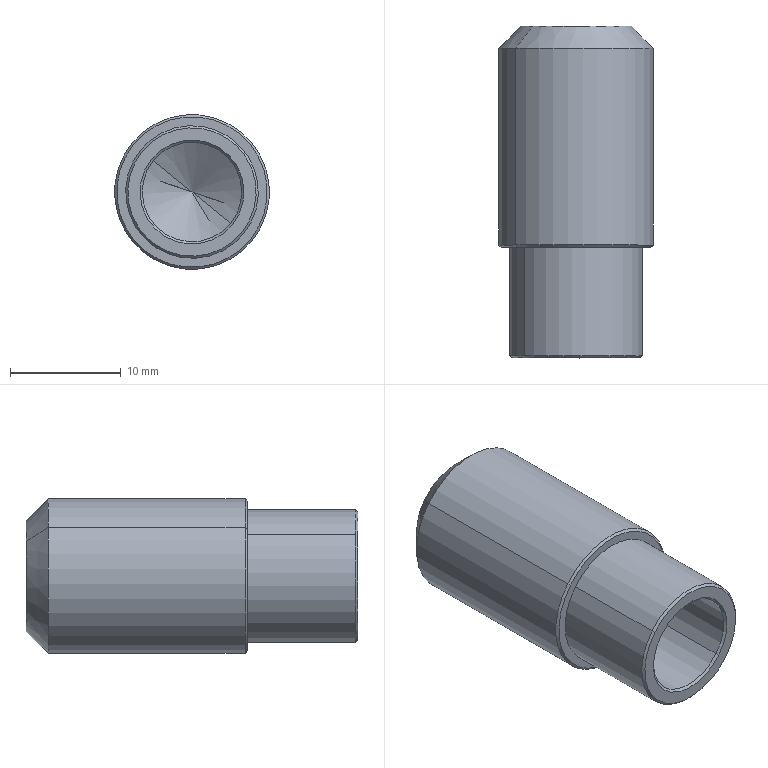Component | SolidWorks | GluePaperFeedingTensioningWheelAssembly-1_YX-04-114GluePaperFeedingTensioningWheelAdjustingPost-1 | 1 solid | 19 faces | box 14 x 30 x 14 mm | volume 2480 mm3 | cone 10 | cylinder 6 | plane 3 | commonest cylinder face diameters 12 x2 14 x2 9 x2 | material 45#Steel
build123d program:
from build123d import *


with BuildPart() as part:
    # Sketch1 → Revolve1 (revolve)
    with BuildSketch(Plane.XY, mode=Mode.PRIVATE) as revolve1_sk:
        Polygon((25, 4.5), (27.704, 0), (30, 0), (30, 5), (28, 7), (10.2, 7), (10, 6.8), (10, 6), (0.2, 6), (0, 5.8), (0, 4.7), (0.2, 4.5), align=None)
    revolve(revolve1_sk.sketch.rotate(Axis((0, 0, 0), (1, 0, 0)), 270), axis=Axis((0, 0, 0), (1, 0, 0)))


solid = part.part

# Placed as in the assembly
solid = solid.moved(Location((16.603, 31.262, 167), (0, 0, 90)))
STEP:
#1=CARTESIAN_POINT('',(0.7915,1.239,6.464));
#2=VERTEX_POINT('',#1);
#3=CARTESIAN_POINT('',(0.5158,1.239,6.686));
#4=VERTEX_POINT('',#3);
#5=CARTESIAN_POINT('',(0.6537,1.239,6.575));
#6=DIRECTION('',(-0.,1.,0.));
#7=DIRECTION('',(-0.778,0.,0.6282));
#8=AXIS2_PLACEMENT_3D('',#5,#6,#7);
#9=CIRCLE('',#8,0.1772);
#10=EDGE_CURVE('',#2,#4,#9,.T.);
#11=ORIENTED_EDGE('',*,*,#10,.T.);
#12=CARTESIAN_POINT('',(0.5097,1.231,6.691));
#13=VERTEX_POINT('',#12);
#14=CARTESIAN_POINT('',(0.5097,1.231,6.691));
#15=DIRECTION('',(-0.5501,-0.7071,0.4442));
#16=VECTOR('',#15,39.37);
#17=LINE('',#14,#16);
#18=EDGE_CURVE('',#4,#13,#17,.T.);
#19=ORIENTED_EDGE('',*,*,#18,.T.);
#20=CARTESIAN_POINT('',(0.7976,1.231,6.459));
#21=VERTEX_POINT('',#20);
#22=CARTESIAN_POINT('',(0.6537,1.231,6.575));
#23=DIRECTION('',(-0.,1.,0.));
#24=DIRECTION('',(-0.778,0.,0.6282));
#25=AXIS2_PLACEMENT_3D('',#22,#23,#24);
#26=CIRCLE('',#25,0.185);
#27=EDGE_CURVE('',#21,#13,#26,.T.);
#28=ORIENTED_EDGE('',*,*,#27,.F.);
#29=CARTESIAN_POINT('',(0.7976,1.231,6.459));
#30=DIRECTION('',(0.5501,-0.7071,-0.4442));
#31=VECTOR('',#30,39.37);
#32=LINE('',#29,#31);
#33=EDGE_CURVE('',#2,#21,#32,.T.);
#34=ORIENTED_EDGE('',*,*,#33,.F.);
#35=EDGE_LOOP('',(#11,#19,#28,#34));
#36=FACE_OUTER_BOUND('',#35,.T.);
#37=CARTESIAN_POINT('',(0.6537,1.231,6.575));
#38=DIRECTION('',(0.,-1.,-0.));
#39=DIRECTION('',(0.778,0.,-0.6282));
#40=AXIS2_PLACEMENT_3D('',#37,#38,#39);
#41=CONICAL_SURFACE('',#40,0.185,0.7854);
#42=ADVANCED_FACE('',(#36),#41,.F.);
#43=CARTESIAN_POINT('',(0.476,1.231,6.718));
#44=VERTEX_POINT('',#43);
#45=CARTESIAN_POINT('',(0.8313,1.231,6.431));
#46=VERTEX_POINT('',#45);
#47=CARTESIAN_POINT('',(0.6537,1.231,6.575));
#48=DIRECTION('',(-0.,1.,0.));
#49=DIRECTION('',(-0.778,0.,0.6282));
#50=AXIS2_PLACEMENT_3D('',#47,#48,#49);
#51=CIRCLE('',#50,0.2283);
#52=EDGE_CURVE('',#44,#46,#51,.T.);
#53=ORIENTED_EDGE('',*,*,#52,.T.);
#54=CARTESIAN_POINT('',(0.8374,1.239,6.426));
#55=VERTEX_POINT('',#54);
#56=CARTESIAN_POINT('',(0.8374,1.239,6.426));
#57=DIRECTION('',(0.5501,0.7071,-0.4442));
#58=VECTOR('',#57,39.37);
#59=LINE('',#56,#58);
#60=EDGE_CURVE('',#46,#55,#59,.T.);
#61=ORIENTED_EDGE('',*,*,#60,.T.);
#62=CARTESIAN_POINT('',(0.4699,1.239,6.723));
#63=VERTEX_POINT('',#62);
#64=CARTESIAN_POINT('',(0.6537,1.239,6.575));
#65=DIRECTION('',(-0.,1.,0.));
#66=DIRECTION('',(-0.778,0.,0.6282));
#67=AXIS2_PLACEMENT_3D('',#64,#65,#66);
#68=CIRCLE('',#67,0.2362);
#69=EDGE_CURVE('',#63,#55,#68,.T.);
#70=ORIENTED_EDGE('',*,*,#69,.F.);
#71=CARTESIAN_POINT('',(0.4699,1.239,6.723));
#72=DIRECTION('',(-0.5501,0.7071,0.4442));
#73=VECTOR('',#72,39.37);
#74=LINE('',#71,#73);
#75=EDGE_CURVE('',#44,#63,#74,.T.);
#76=ORIENTED_EDGE('',*,*,#75,.F.);
#77=EDGE_LOOP('',(#53,#61,#70,#76));
#78=FACE_OUTER_BOUND('',#77,.T.);
#79=CARTESIAN_POINT('',(0.6537,1.239,6.575));
#80=DIRECTION('',(-0.,1.,0.));
#81=DIRECTION('',(-0.778,0.,0.6282));
#82=AXIS2_PLACEMENT_3D('',#79,#80,#81);
#83=CONICAL_SURFACE('',#82,0.2362,0.7854);
#84=ADVANCED_FACE('',(#78),#83,.T.);
#85=ORIENTED_EDGE('',*,*,#69,.T.);
#86=CARTESIAN_POINT('',(0.8374,1.624,6.426));
#87=VERTEX_POINT('',#86);
#88=CARTESIAN_POINT('',(0.8374,1.231,6.426));
#89=DIRECTION('',(-0.,1.,0.));
#90=VECTOR('',#89,39.37);
#91=LINE('',#88,#90);
#92=EDGE_CURVE('',#55,#87,#91,.T.);
#93=ORIENTED_EDGE('',*,*,#92,.T.);
#94=CARTESIAN_POINT('',(0.4699,1.624,6.723));
#95=VERTEX_POINT('',#94);
#96=CARTESIAN_POINT('',(0.6537,1.624,6.575));
#97=DIRECTION('',(-0.,1.,0.));
#98=DIRECTION('',(-0.778,0.,0.6282));
#99=AXIS2_PLACEMENT_3D('',#96,#97,#98);
#100=CIRCLE('',#99,0.2362);
#101=EDGE_CURVE('',#95,#87,#100,.T.);
#102=ORIENTED_EDGE('',*,*,#101,.F.);
#103=CARTESIAN_POINT('',(0.4699,1.231,6.723));
#104=DIRECTION('',(-0.,1.,0.));
#105=VECTOR('',#104,39.37);
#106=LINE('',#103,#105);
#107=EDGE_CURVE('',#63,#95,#106,.T.);
#108=ORIENTED_EDGE('',*,*,#107,.F.);
#109=EDGE_LOOP('',(#85,#93,#102,#108));
#110=FACE_OUTER_BOUND('',#109,.T.);
#111=CARTESIAN_POINT('',(0.6537,1.231,6.575));
#112=DIRECTION('',(-0.,1.,0.));
#113=DIRECTION('',(-0.778,0.,0.6282));
#114=AXIS2_PLACEMENT_3D('',#111,#112,#113);
#115=CYLINDRICAL_SURFACE('',#114,0.2362);
#116=ADVANCED_FACE('',(#110),#115,.T.);
#117=CARTESIAN_POINT('',(0.4454,1.624,6.743));
#118=VERTEX_POINT('',#117);
#119=CARTESIAN_POINT('',(0.8619,1.624,6.407));
#120=VERTEX_POINT('',#119);
#121=CARTESIAN_POINT('',(0.6537,1.624,6.575));
#122=DIRECTION('',(-0.,1.,0.));
#123=DIRECTION('',(-0.778,0.,0.6282));
#124=AXIS2_PLACEMENT_3D('',#121,#122,#123);
#125=CIRCLE('',#124,0.2677);
#126=EDGE_CURVE('',#118,#120,#125,.T.);
#127=ORIENTED_EDGE('',*,*,#126,.T.);
#128=CARTESIAN_POINT('',(0.8681,1.632,6.402));
#129=VERTEX_POINT('',#128);
#130=CARTESIAN_POINT('',(0.8681,1.632,6.402));
#131=DIRECTION('',(0.5501,0.7071,-0.4442));
#132=VECTOR('',#131,39.37);
#133=LINE('',#130,#132);
#134=EDGE_CURVE('',#120,#129,#133,.T.);
#135=ORIENTED_EDGE('',*,*,#134,.T.);
#136=CARTESIAN_POINT('',(0.4392,1.632,6.748));
#137=VERTEX_POINT('',#136);
#138=CARTESIAN_POINT('',(0.6537,1.632,6.575));
#139=DIRECTION('',(-0.,1.,0.));
#140=DIRECTION('',(-0.778,0.,0.6282));
#141=AXIS2_PLACEMENT_3D('',#138,#139,#140);
#142=CIRCLE('',#141,0.2756);
#143=EDGE_CURVE('',#137,#129,#142,.T.);
#144=ORIENTED_EDGE('',*,*,#143,.F.);
#145=CARTESIAN_POINT('',(0.4392,1.632,6.748));
#146=DIRECTION('',(-0.5501,0.7071,0.4442));
#147=VECTOR('',#146,39.37);
#148=LINE('',#145,#147);
#149=EDGE_CURVE('',#118,#137,#148,.T.);
#150=ORIENTED_EDGE('',*,*,#149,.F.);
#151=EDGE_LOOP('',(#127,#135,#144,#150));
#152=FACE_OUTER_BOUND('',#151,.T.);
#153=CARTESIAN_POINT('',(0.6537,1.632,6.575));
#154=DIRECTION('',(-0.,1.,0.));
#155=DIRECTION('',(-0.778,0.,0.6282));
#156=AXIS2_PLACEMENT_3D('',#153,#154,#155);
#157=CONICAL_SURFACE('',#156,0.2756,0.7854);
#158=ADVANCED_FACE('',(#152),#157,.T.);
#159=ORIENTED_EDGE('',*,*,#143,.T.);
#160=CARTESIAN_POINT('',(0.8681,2.333,6.402));
#161=VERTEX_POINT('',#160);
#162=CARTESIAN_POINT('',(0.8681,1.231,6.402));
#163=DIRECTION('',(-0.,1.,0.));
#164=VECTOR('',#163,39.37);
#165=LINE('',#162,#164);
#166=EDGE_CURVE('',#129,#161,#165,.T.);
#167=ORIENTED_EDGE('',*,*,#166,.T.);
#168=CARTESIAN_POINT('',(0.4392,2.333,6.748));
#169=VERTEX_POINT('',#168);
#170=CARTESIAN_POINT('',(0.6537,2.333,6.575));
#171=DIRECTION('',(-0.,1.,0.));
#172=DIRECTION('',(-0.778,0.,0.6282));
#173=AXIS2_PLACEMENT_3D('',#170,#171,#172);
#174=CIRCLE('',#173,0.2756);
#175=EDGE_CURVE('',#169,#161,#174,.T.);
#176=ORIENTED_EDGE('',*,*,#175,.F.);
#177=CARTESIAN_POINT('',(0.4392,1.231,6.748));
#178=DIRECTION('',(-0.,1.,0.));
#179=VECTOR('',#178,39.37);
#180=LINE('',#177,#179);
#181=EDGE_CURVE('',#137,#169,#180,.T.);
#182=ORIENTED_EDGE('',*,*,#181,.F.);
#183=EDGE_LOOP('',(#159,#167,#176,#182));
#184=FACE_OUTER_BOUND('',#183,.T.);
#185=CARTESIAN_POINT('',(0.6537,1.231,6.575));
#186=DIRECTION('',(-0.,1.,0.));
#187=DIRECTION('',(-0.778,0.,0.6282));
#188=AXIS2_PLACEMENT_3D('',#185,#186,#187);
#189=CYLINDRICAL_SURFACE('',#188,0.2756);
#190=ADVANCED_FACE('',(#184),#189,.T.);
#191=CARTESIAN_POINT('',(0.5005,2.412,6.698));
#192=VERTEX_POINT('',#191);
#193=CARTESIAN_POINT('',(0.8068,2.412,6.451));
#194=VERTEX_POINT('',#193);
#195=CARTESIAN_POINT('',(0.6537,2.412,6.575));
#196=DIRECTION('',(-0.,1.,0.));
#197=DIRECTION('',(-0.778,0.,0.6282));
#198=AXIS2_PLACEMENT_3D('',#195,#196,#197);
#199=CIRCLE('',#198,0.1969);
#200=EDGE_CURVE('',#192,#194,#199,.T.);
#201=ORIENTED_EDGE('',*,*,#200,.F.);
#202=CARTESIAN_POINT('',(0.5005,2.412,6.698));
#203=DIRECTION('',(-0.5501,-0.7071,0.4442));
#204=VECTOR('',#203,39.37);
#205=LINE('',#202,#204);
#206=EDGE_CURVE('',#192,#169,#205,.T.);
#207=ORIENTED_EDGE('',*,*,#206,.T.);
#208=ORIENTED_EDGE('',*,*,#175,.T.);
#209=CARTESIAN_POINT('',(0.8068,2.412,6.451));
#210=DIRECTION('',(0.5501,-0.7071,-0.4442));
#211=VECTOR('',#210,39.37);
#212=LINE('',#209,#211);
#213=EDGE_CURVE('',#194,#161,#212,.T.);
#214=ORIENTED_EDGE('',*,*,#213,.F.);
#215=EDGE_LOOP('',(#201,#207,#208,#214));
#216=FACE_OUTER_BOUND('',#215,.T.);
#217=CARTESIAN_POINT('',(0.6537,2.412,6.575));
#218=DIRECTION('',(0.,-1.,-0.));
#219=DIRECTION('',(0.778,0.,-0.6282));
#220=AXIS2_PLACEMENT_3D('',#217,#218,#219);
#221=CONICAL_SURFACE('',#220,0.1969,0.7854);
#222=ADVANCED_FACE('',(#216),#221,.T.);
#223=CARTESIAN_POINT('',(0.6537,2.321,6.575));
#224=VERTEX_POINT('',#223);
#225=CARTESIAN_POINT('',(0.7915,2.215,6.464));
#226=VERTEX_POINT('',#225);
#227=CARTESIAN_POINT('',(0.7915,2.215,6.464));
#228=DIRECTION('',(0.6669,-0.515,-0.5385));
#229=VECTOR('',#228,39.37);
#230=LINE('',#227,#229);
#231=EDGE_CURVE('',#224,#226,#230,.T.);
#232=ORIENTED_EDGE('',*,*,#231,.F.);
#233=CARTESIAN_POINT('',(0.5158,2.215,6.686));
#234=VERTEX_POINT('',#233);
#235=CARTESIAN_POINT('',(0.5158,2.215,6.686));
#236=DIRECTION('',(-0.6669,-0.515,0.5385));
#237=VECTOR('',#236,39.37);
#238=LINE('',#235,#237);
#239=EDGE_CURVE('',#224,#234,#238,.T.);
#240=ORIENTED_EDGE('',*,*,#239,.T.);
#241=CARTESIAN_POINT('',(0.6537,2.215,6.575));
#242=DIRECTION('',(-0.,1.,0.));
#243=DIRECTION('',(-0.778,0.,0.6282));
#244=AXIS2_PLACEMENT_3D('',#241,#242,#243);
#245=CIRCLE('',#244,0.1772);
#246=EDGE_CURVE('',#226,#234,#245,.T.);
#247=ORIENTED_EDGE('',*,*,#246,.F.);
#248=EDGE_LOOP('',(#232,#240,#247));
#249=FACE_OUTER_BOUND('',#248,.T.);
#250=CARTESIAN_POINT('',(0.6537,2.215,6.575));
#251=DIRECTION('',(0.,-1.,-0.));
#252=DIRECTION('',(0.778,0.,-0.6282));
#253=AXIS2_PLACEMENT_3D('',#250,#251,#252);
#254=CONICAL_SURFACE('',#253,0.1772,1.03);
#255=ADVANCED_FACE('',(#249),#254,.F.);
#256=ORIENTED_EDGE('',*,*,#10,.F.);
#257=CARTESIAN_POINT('',(0.7915,1.231,6.464));
#258=DIRECTION('',(-0.,1.,0.));
#259=VECTOR('',#258,39.37);
#260=LINE('',#257,#259);
#261=EDGE_CURVE('',#2,#226,#260,.T.);
#262=ORIENTED_EDGE('',*,*,#261,.T.);
#263=ORIENTED_EDGE('',*,*,#246,.T.);
#264=CARTESIAN_POINT('',(0.5158,1.231,6.686));
#265=DIRECTION('',(-0.,1.,0.));
#266=VECTOR('',#265,39.37);
#267=LINE('',#264,#266);
#268=EDGE_CURVE('',#4,#234,#267,.T.);
#269=ORIENTED_EDGE('',*,*,#268,.F.);
#270=EDGE_LOOP('',(#256,#262,#263,#269));
#271=FACE_OUTER_BOUND('',#270,.T.);
#272=CARTESIAN_POINT('',(0.6537,1.231,6.575));
#273=DIRECTION('',(-0.,1.,0.));
#274=DIRECTION('',(-0.778,0.,0.6282));
#275=AXIS2_PLACEMENT_3D('',#272,#273,#274);
#276=CYLINDRICAL_SURFACE('',#275,0.1772);
#277=ADVANCED_FACE('',(#271),#276,.F.);
#278=ORIENTED_EDGE('',*,*,#261,.F.);
#279=CARTESIAN_POINT('',(0.6537,1.239,6.575));
#280=DIRECTION('',(-0.,1.,0.));
#281=DIRECTION('',(-0.778,0.,0.6282));
#282=AXIS2_PLACEMENT_3D('',#279,#280,#281);
#283=CIRCLE('',#282,0.1772);
#284=EDGE_CURVE('',#4,#2,#283,.T.);
#285=ORIENTED_EDGE('',*,*,#284,.F.);
#286=ORIENTED_EDGE('',*,*,#268,.T.);
#287=CARTESIAN_POINT('',(0.6537,2.215,6.575));
#288=DIRECTION('',(-0.,1.,0.));
#289=DIRECTION('',(-0.778,0.,0.6282));
#290=AXIS2_PLACEMENT_3D('',#287,#288,#289);
#291=CIRCLE('',#290,0.1772);
#292=EDGE_CURVE('',#234,#226,#291,.T.);
#293=ORIENTED_EDGE('',*,*,#292,.T.);
#294=EDGE_LOOP('',(#278,#285,#286,#293));
#295=FACE_OUTER_BOUND('',#294,.T.);
#296=CARTESIAN_POINT('',(0.6537,1.231,6.575));
#297=DIRECTION('',(-0.,1.,0.));
#298=DIRECTION('',(-0.778,0.,0.6282));
#299=AXIS2_PLACEMENT_3D('',#296,#297,#298);
#300=CYLINDRICAL_SURFACE('',#299,0.1772);
#301=ADVANCED_FACE('',(#295),#300,.F.);
#302=ORIENTED_EDGE('',*,*,#239,.F.);
#303=ORIENTED_EDGE('',*,*,#231,.T.);
#304=ORIENTED_EDGE('',*,*,#292,.F.);
#305=EDGE_LOOP('',(#302,#303,#304));
#306=FACE_OUTER_BOUND('',#305,.T.);
#307=CARTESIAN_POINT('',(0.6537,2.215,6.575));
#308=DIRECTION('',(0.,-1.,-0.));
#309=DIRECTION('',(0.778,0.,-0.6282));
#310=AXIS2_PLACEMENT_3D('',#307,#308,#309);
#311=CONICAL_SURFACE('',#310,0.1772,1.03);
#312=ADVANCED_FACE('',(#306),#311,.F.);
#313=CARTESIAN_POINT('',(0.6537,2.412,6.575));
#314=DIRECTION('',(-0.,1.,0.));
#315=DIRECTION('',(-0.778,0.,0.6282));
#316=AXIS2_PLACEMENT_3D('',#313,#314,#315);
#317=CIRCLE('',#316,0.1969);
#318=EDGE_CURVE('',#194,#192,#317,.T.);
#319=ORIENTED_EDGE('',*,*,#318,.T.);
#320=ORIENTED_EDGE('',*,*,#200,.T.);
#321=EDGE_LOOP('',(#319,#320));
#322=FACE_OUTER_BOUND('',#321,.T.);
#323=CARTESIAN_POINT('',(0.6537,2.412,6.575));
#324=DIRECTION('',(-0.,1.,0.));
#325=DIRECTION('',(-0.778,-0.,0.6282));
#326=AXIS2_PLACEMENT_3D('',#323,#324,#325);
#327=PLANE('',#326);
#328=ADVANCED_FACE('',(#322),#327,.T.);
#329=ORIENTED_EDGE('',*,*,#206,.F.);
#330=ORIENTED_EDGE('',*,*,#318,.F.);
#331=ORIENTED_EDGE('',*,*,#213,.T.);
#332=CARTESIAN_POINT('',(0.6537,2.333,6.575));
#333=DIRECTION('',(-0.,1.,0.));
#334=DIRECTION('',(-0.778,0.,0.6282));
#335=AXIS2_PLACEMENT_3D('',#332,#333,#334);
#336=CIRCLE('',#335,0.2756);
#337=EDGE_CURVE('',#161,#169,#336,.T.);
#338=ORIENTED_EDGE('',*,*,#337,.T.);
#339=EDGE_LOOP('',(#329,#330,#331,#338));
#340=FACE_OUTER_BOUND('',#339,.T.);
#341=CARTESIAN_POINT('',(0.6537,2.412,6.575));
#342=DIRECTION('',(0.,-1.,-0.));
#343=DIRECTION('',(0.778,0.,-0.6282));
#344=AXIS2_PLACEMENT_3D('',#341,#342,#343);
#345=CONICAL_SURFACE('',#344,0.1969,0.7854);
#346=ADVANCED_FACE('',(#340),#345,.T.);
#347=ORIENTED_EDGE('',*,*,#166,.F.);
#348=CARTESIAN_POINT('',(0.6537,1.632,6.575));
#349=DIRECTION('',(-0.,1.,0.));
#350=DIRECTION('',(-0.778,0.,0.6282));
#351=AXIS2_PLACEMENT_3D('',#348,#349,#350);
#352=CIRCLE('',#351,0.2756);
#353=EDGE_CURVE('',#129,#137,#352,.T.);
#354=ORIENTED_EDGE('',*,*,#353,.T.);
#355=ORIENTED_EDGE('',*,*,#181,.T.);
#356=ORIENTED_EDGE('',*,*,#337,.F.);
#357=EDGE_LOOP('',(#347,#354,#355,#356));
#358=FACE_OUTER_BOUND('',#357,.T.);
#359=CARTESIAN_POINT('',(0.6537,1.231,6.575));
#360=DIRECTION('',(-0.,1.,0.));
#361=DIRECTION('',(-0.778,0.,0.6282));
#362=AXIS2_PLACEMENT_3D('',#359,#360,#361);
#363=CYLINDRICAL_SURFACE('',#362,0.2756);
#364=ADVANCED_FACE('',(#358),#363,.T.);
#365=ORIENTED_EDGE('',*,*,#134,.F.);
#366=CARTESIAN_POINT('',(0.6537,1.624,6.575));
#367=DIRECTION('',(-0.,1.,0.));
#368=DIRECTION('',(-0.778,0.,0.6282));
#369=AXIS2_PLACEMENT_3D('',#366,#367,#368);
#370=CIRCLE('',#369,0.2677);
#371=EDGE_CURVE('',#120,#118,#370,.T.);
#372=ORIENTED_EDGE('',*,*,#371,.T.);
#373=ORIENTED_EDGE('',*,*,#149,.T.);
#374=ORIENTED_EDGE('',*,*,#353,.F.);
#375=EDGE_LOOP('',(#365,#372,#373,#374));
#376=FACE_OUTER_BOUND('',#375,.T.);
#377=CARTESIAN_POINT('',(0.6537,1.632,6.575));
#378=DIRECTION('',(-0.,1.,0.));
#379=DIRECTION('',(-0.778,0.,0.6282));
#380=AXIS2_PLACEMENT_3D('',#377,#378,#379);
#381=CONICAL_SURFACE('',#380,0.2756,0.7854);
#382=ADVANCED_FACE('',(#376),#381,.T.);
#383=ORIENTED_EDGE('',*,*,#101,.T.);
#384=CARTESIAN_POINT('',(0.6537,1.624,6.575));
#385=DIRECTION('',(-0.,1.,0.));
#386=DIRECTION('',(-0.778,0.,0.6282));
#387=AXIS2_PLACEMENT_3D('',#384,#385,#386);
#388=CIRCLE('',#387,0.2362);
#389=EDGE_CURVE('',#87,#95,#388,.T.);
#390=ORIENTED_EDGE('',*,*,#389,.T.);
#391=EDGE_LOOP('',(#383,#390));
#392=FACE_BOUND('',#391,.T.);
#393=ORIENTED_EDGE('',*,*,#126,.F.);
#394=ORIENTED_EDGE('',*,*,#371,.F.);
#395=EDGE_LOOP('',(#393,#394));
#396=FACE_OUTER_BOUND('',#395,.T.);
#397=CARTESIAN_POINT('',(0.8218,1.624,6.783));
#398=DIRECTION('',(0.,-1.,-0.));
#399=DIRECTION('',(0.778,0.,-0.6282));
#400=AXIS2_PLACEMENT_3D('',#397,#398,#399);
#401=PLANE('',#400);
#402=ADVANCED_FACE('',(#392,#396),#401,.T.);
#403=ORIENTED_EDGE('',*,*,#92,.F.);
#404=CARTESIAN_POINT('',(0.6537,1.239,6.575));
#405=DIRECTION('',(-0.,1.,0.));
#406=DIRECTION('',(-0.778,0.,0.6282));
#407=AXIS2_PLACEMENT_3D('',#404,#405,#406);
#408=CIRCLE('',#407,0.2362);
#409=EDGE_CURVE('',#55,#63,#408,.T.);
#410=ORIENTED_EDGE('',*,*,#409,.T.);
#411=ORIENTED_EDGE('',*,*,#107,.T.);
#412=ORIENTED_EDGE('',*,*,#389,.F.);
#413=EDGE_LOOP('',(#403,#410,#411,#412));
#414=FACE_OUTER_BOUND('',#413,.T.);
#415=CARTESIAN_POINT('',(0.6537,1.231,6.575));
#416=DIRECTION('',(-0.,1.,0.));
#417=DIRECTION('',(-0.778,0.,0.6282));
#418=AXIS2_PLACEMENT_3D('',#415,#416,#417);
#419=CYLINDRICAL_SURFACE('',#418,0.2362);
#420=ADVANCED_FACE('',(#414),#419,.T.);
#421=ORIENTED_EDGE('',*,*,#60,.F.);
#422=CARTESIAN_POINT('',(0.6537,1.231,6.575));
#423=DIRECTION('',(-0.,1.,0.));
#424=DIRECTION('',(-0.778,0.,0.6282));
#425=AXIS2_PLACEMENT_3D('',#422,#423,#424);
#426=CIRCLE('',#425,0.2283);
#427=EDGE_CURVE('',#46,#44,#426,.T.);
#428=ORIENTED_EDGE('',*,*,#427,.T.);
#429=ORIENTED_EDGE('',*,*,#75,.T.);
#430=ORIENTED_EDGE('',*,*,#409,.F.);
#431=EDGE_LOOP('',(#421,#428,#429,#430));
#432=FACE_OUTER_BOUND('',#431,.T.);
#433=CARTESIAN_POINT('',(0.6537,1.239,6.575));
#434=DIRECTION('',(-0.,1.,0.));
#435=DIRECTION('',(-0.778,0.,0.6282));
#436=AXIS2_PLACEMENT_3D('',#433,#434,#435);
#437=CONICAL_SURFACE('',#436,0.2362,0.7854);
#438=ADVANCED_FACE('',(#432),#437,.T.);
#439=ORIENTED_EDGE('',*,*,#27,.T.);
#440=CARTESIAN_POINT('',(0.6537,1.231,6.575));
#441=DIRECTION('',(-0.,1.,0.));
#442=DIRECTION('',(-0.778,0.,0.6282));
#443=AXIS2_PLACEMENT_3D('',#440,#441,#442);
#444=CIRCLE('',#443,0.185);
#445=EDGE_CURVE('',#13,#21,#444,.T.);
#446=ORIENTED_EDGE('',*,*,#445,.T.);
#447=EDGE_LOOP('',(#439,#446));
#448=FACE_BOUND('',#447,.T.);
#449=ORIENTED_EDGE('',*,*,#52,.F.);
#450=ORIENTED_EDGE('',*,*,#427,.F.);
#451=EDGE_LOOP('',(#449,#450));
#452=FACE_OUTER_BOUND('',#451,.T.);
#453=CARTESIAN_POINT('',(0.7971,1.231,6.752));
#454=DIRECTION('',(0.,-1.,-0.));
#455=DIRECTION('',(0.778,0.,-0.6282));
#456=AXIS2_PLACEMENT_3D('',#453,#454,#455);
#457=PLANE('',#456);
#458=ADVANCED_FACE('',(#448,#452),#457,.T.);
#459=ORIENTED_EDGE('',*,*,#18,.F.);
#460=ORIENTED_EDGE('',*,*,#284,.T.);
#461=ORIENTED_EDGE('',*,*,#33,.T.);
#462=ORIENTED_EDGE('',*,*,#445,.F.);
#463=EDGE_LOOP('',(#459,#460,#461,#462));
#464=FACE_OUTER_BOUND('',#463,.T.);
#465=CARTESIAN_POINT('',(0.6537,1.231,6.575));
#466=DIRECTION('',(0.,-1.,-0.));
#467=DIRECTION('',(0.778,0.,-0.6282));
#468=AXIS2_PLACEMENT_3D('',#465,#466,#467);
#469=CONICAL_SURFACE('',#468,0.185,0.7854);
#470=ADVANCED_FACE('',(#464),#469,.F.);
#471=CLOSED_SHELL('',(#42,#84,#116,#158,#190,#222,#255,#277,#301,#312,#328,#346,#364,#382,#402,#420,#438,#458,#470));
#472=MANIFOLD_SOLID_BREP('',#471);
#473=CARTESIAN_POINT('',(0.,0.,0.));
#474=DIRECTION('',(0.,0.,1.));
#475=DIRECTION('',(1.,0.,0.));
#476=AXIS2_PLACEMENT_3D('',#473,#474,#475);
#477=(LENGTH_UNIT()NAMED_UNIT(*)SI_UNIT($,.METRE.));
#478=LENGTH_MEASURE_WITH_UNIT(LENGTH_MEASURE(0.0254),#477);
#479=DIMENSIONAL_EXPONENTS(1.,0.,0.,0.,0.,0.,0.);
#480=(CONVERSION_BASED_UNIT('',#478)LENGTH_UNIT()NAMED_UNIT(#479));
#481=UNCERTAINTY_MEASURE_WITH_UNIT(LENGTH_MEASURE(0.00001),#480,'','');
#482=(NAMED_UNIT(*)PLANE_ANGLE_UNIT()SI_UNIT($,.RADIAN.));
#483=(NAMED_UNIT(*)SI_UNIT($,.STERADIAN.)SOLID_ANGLE_UNIT());
#484=(GEOMETRIC_REPRESENTATION_CONTEXT(3)GLOBAL_UNCERTAINTY_ASSIGNED_CONTEXT((#481))GLOBAL_UNIT_ASSIGNED_CONTEXT((#480,#482,#483))REPRESENTATION_CONTEXT('',''));
#485=ADVANCED_BREP_SHAPE_REPRESENTATION('',(#472,#476),#484);
#486=COLOUR_RGB('',0.7922,0.8196,0.9333);
#487=FILL_AREA_STYLE_COLOUR('',#486);
#488=FILL_AREA_STYLE('',(#487));
#489=SURFACE_STYLE_FILL_AREA(#488);
#490=SURFACE_SIDE_STYLE('',(#489));
#491=SURFACE_STYLE_USAGE(.BOTH.,#490);
#492=PRESENTATION_STYLE_ASSIGNMENT((#491));
#493=STYLED_ITEM('',(#492),#472);
#494=(LENGTH_UNIT()NAMED_UNIT(*)SI_UNIT($,.METRE.));
#495=LENGTH_MEASURE_WITH_UNIT(LENGTH_MEASURE(0.0254),#494);
#496=DIMENSIONAL_EXPONENTS(1.,0.,0.,0.,0.,0.,0.);
#497=(CONVERSION_BASED_UNIT('',#495)LENGTH_UNIT()NAMED_UNIT(#496));
#498=UNCERTAINTY_MEASURE_WITH_UNIT(LENGTH_MEASURE(0.00001),#497,'','');
#499=(NAMED_UNIT(*)PLANE_ANGLE_UNIT()SI_UNIT($,.RADIAN.));
#500=(NAMED_UNIT(*)SI_UNIT($,.STERADIAN.)SOLID_ANGLE_UNIT());
#501=(GEOMETRIC_REPRESENTATION_CONTEXT(3)GLOBAL_UNCERTAINTY_ASSIGNED_CONTEXT((#498))GLOBAL_UNIT_ASSIGNED_CONTEXT((#497,#499,#500))REPRESENTATION_CONTEXT('',''));
#502=MECHANICAL_DESIGN_GEOMETRIC_PRESENTATION_REPRESENTATION('',(#493),#501);
#503=PRESENTATION_LAYER_ASSIGNMENT('','',(#493));